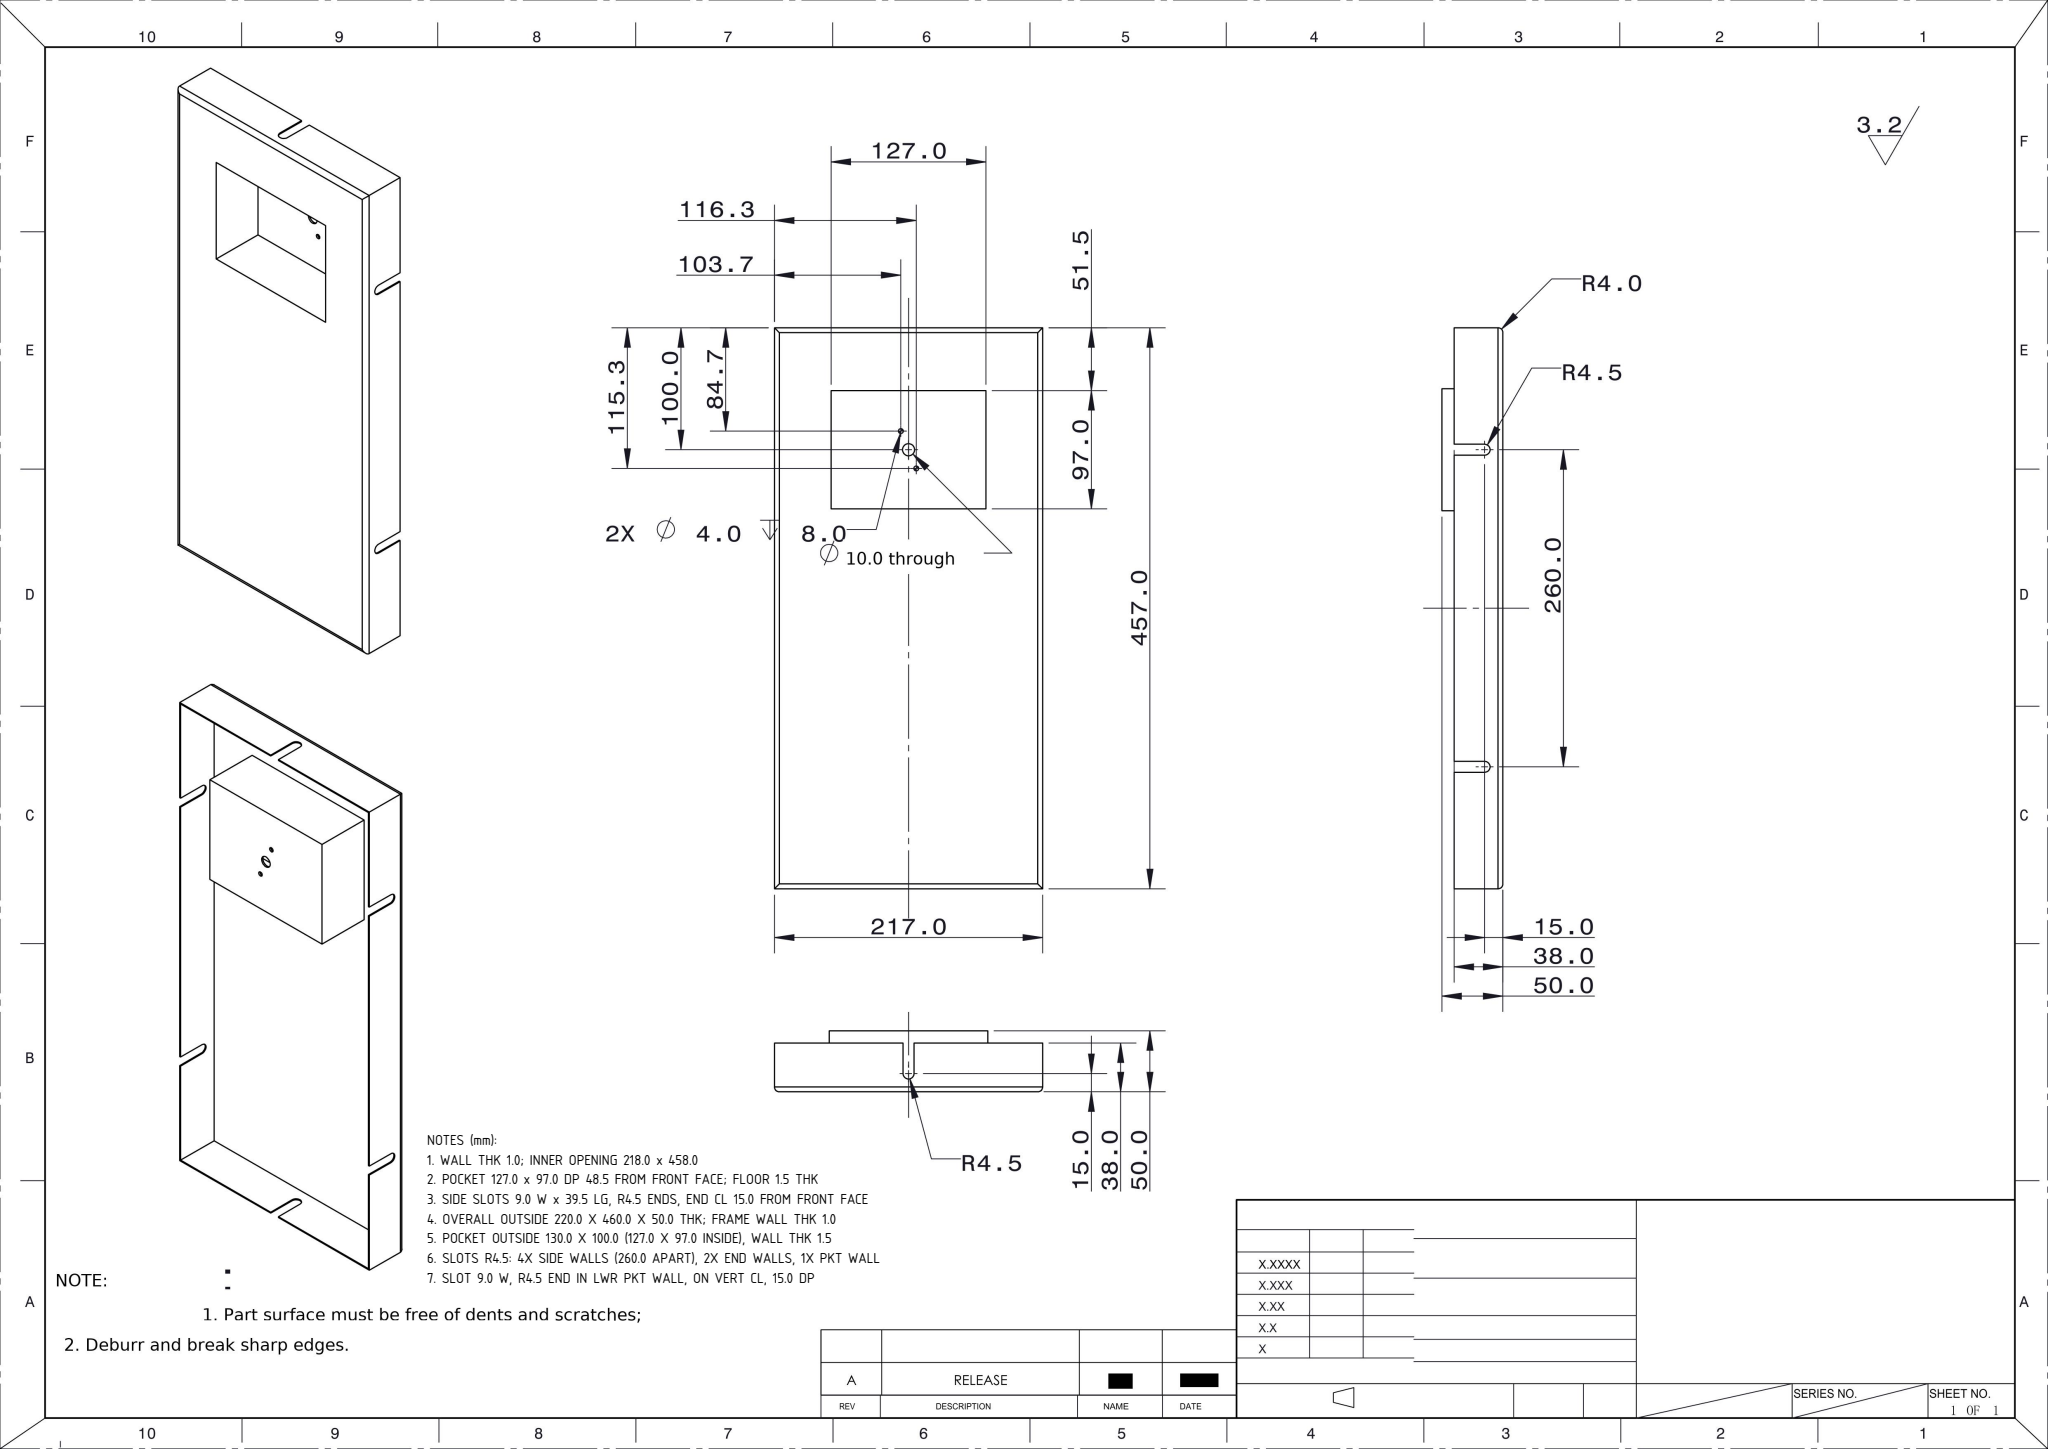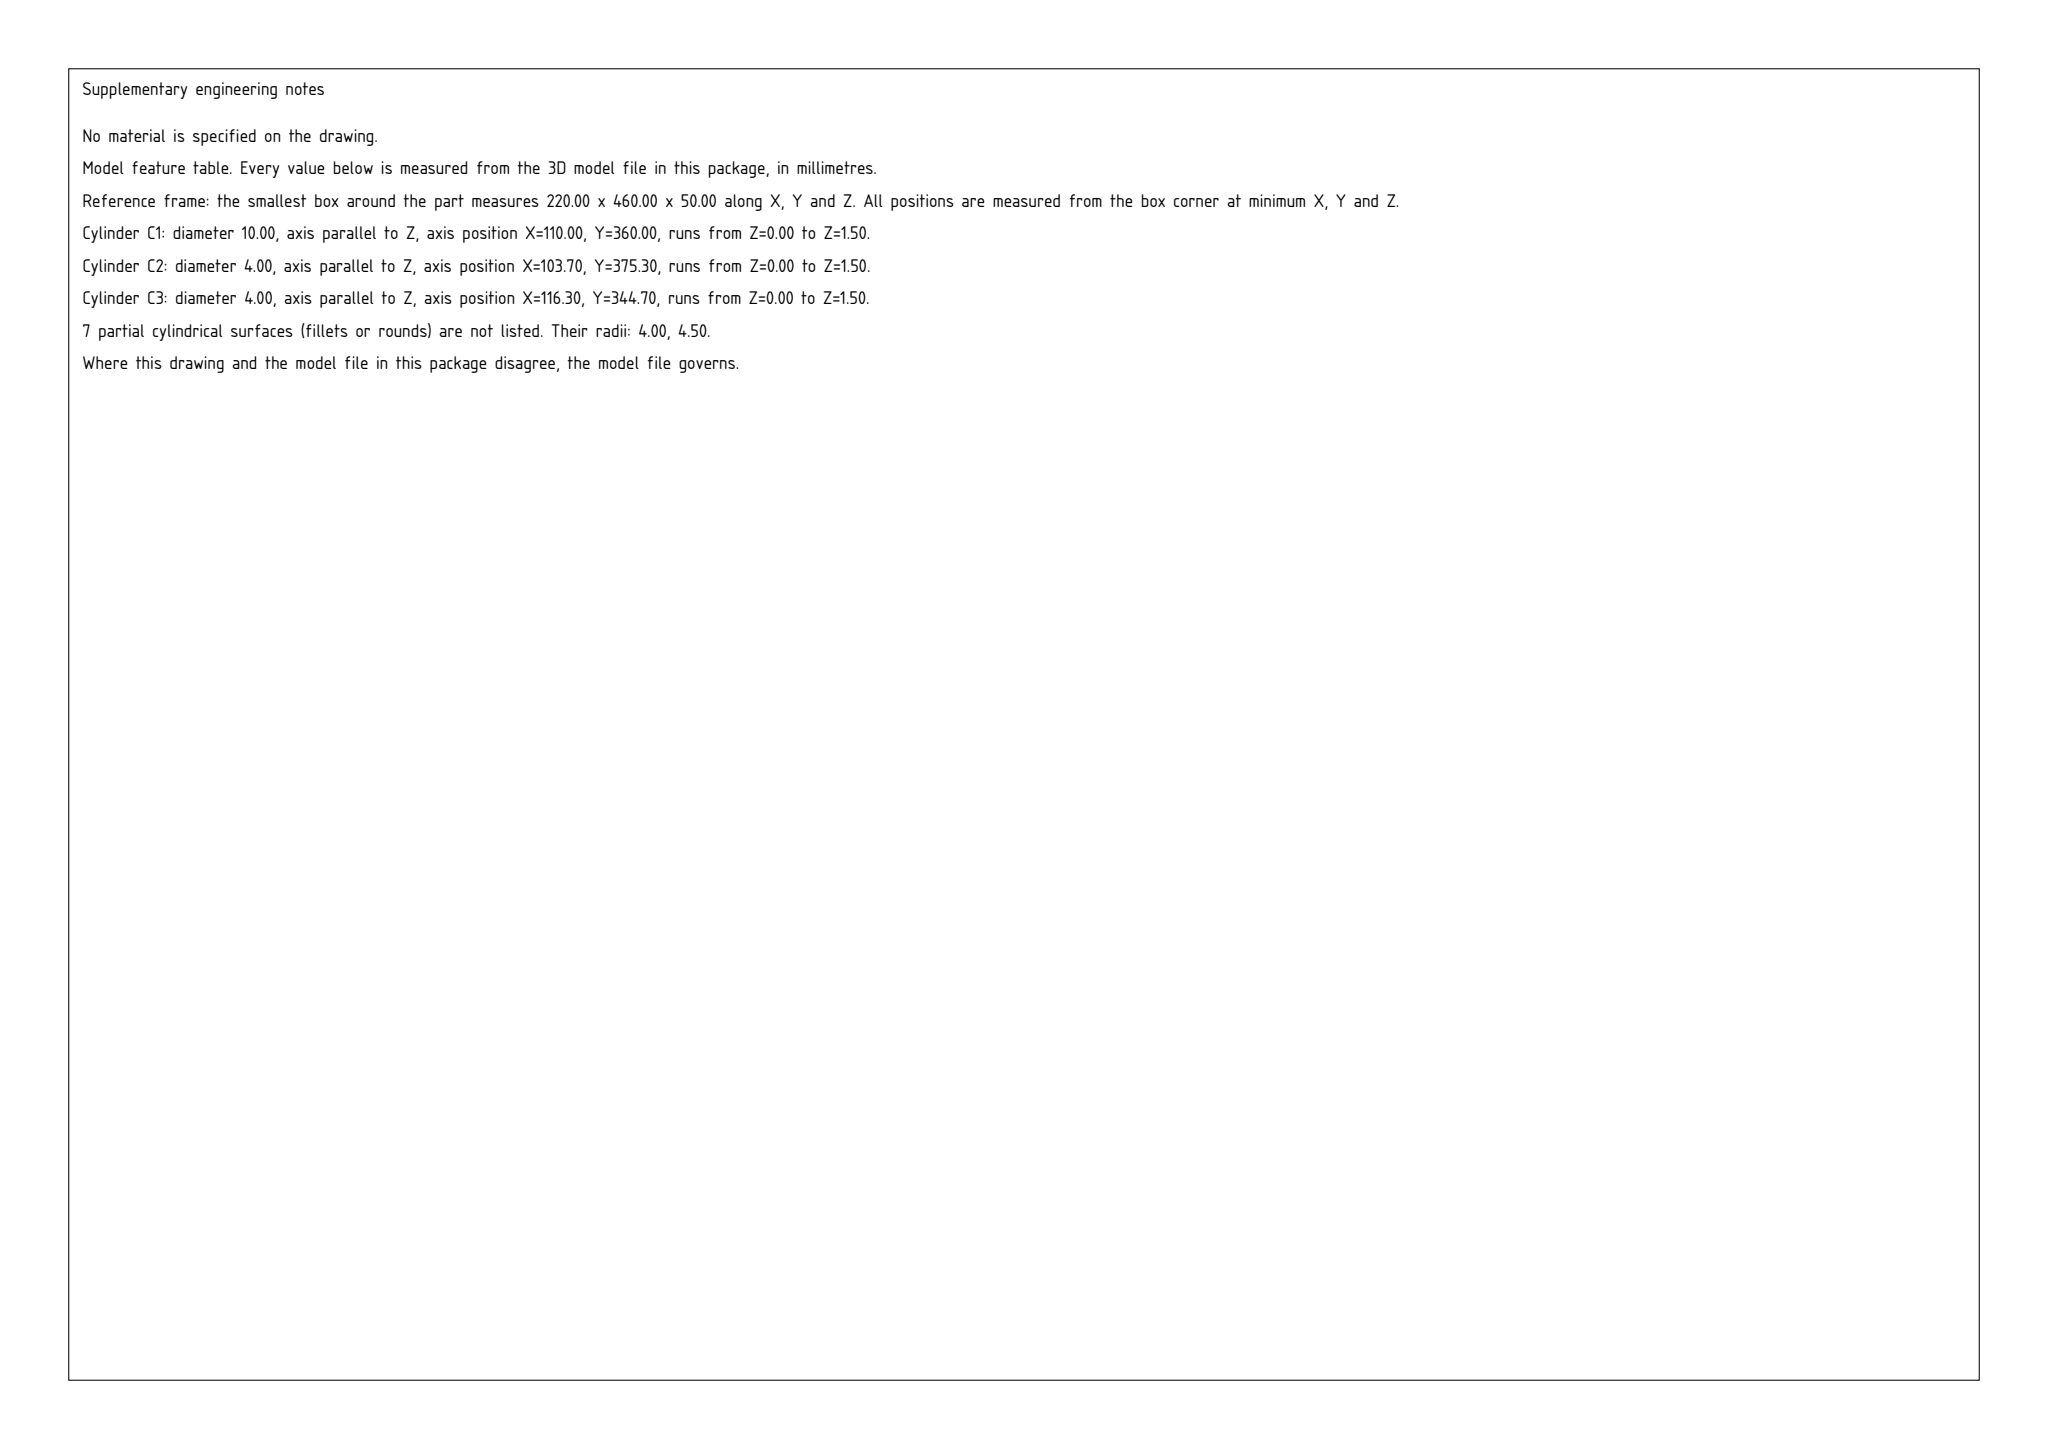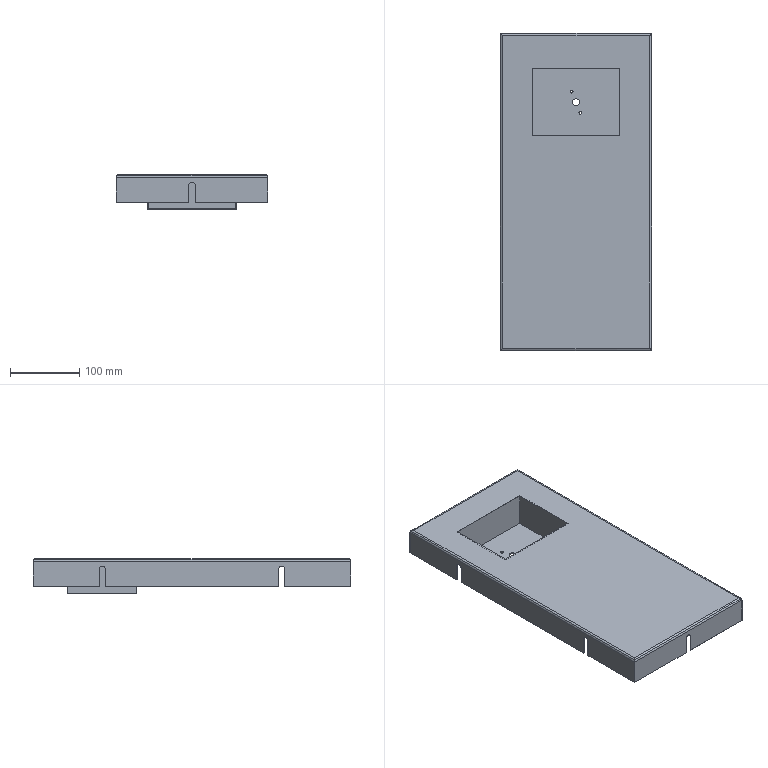Part | SolidWorks | mm | 1 solid | 55 faces | box 220 x 460 x 50 mm | volume 187271 mm3 | plane 38 | cylinder 17 | commonest cylinder face diameters 9 x7 4 x4 8 x4 10 x2
Drawing notes:
WALL THK 1.0; INNER OPENING 218.0 x 458.0 | from the solid: x-planes 0/1 & 219/220, y-planes 0/1 & 459/460 -> 1.0 wall, inner 218.0 x 458.0
POCKET 127.0 x 97.0 DP 48.5 FROM FRONT FACE; FLOOR 1.5 THK | from the solid: pocket inner x 46.5-173.5 (127.0), y 311.5-408.5 (97.0); floor z 0-1.5; front face z=50
SIDE SLOTS 9.0 W x 39.5 LG, R4.5 ENDS, END CL 15.0 FROM FRONT FACE | from the solid: O9 x-axis cyls at y=100 & y=360, z=35 thru 1.0 wall; y-planes 95.5/104.5; z 0-39.5; 50-35=15.0
OVERALL OUTSIDE 220.0 X 460.0 X 50.0 THK; FRAME WALL THK 1.0 | from the solid: bbox_xyz 220.0x460.0x50.0; x planes 0/1.0 & 219.0/220.0, y planes 0/1.0 & 459.0/460.0 give 1.0 wall
POCKET OUTSIDE 130.0 X 100.0 (127.0 X 97.0 INSIDE), WALL THK 1.5 | from the solid: x planes 45.0 & 175.0 (outside) vs 46.5 & 173.5 (inside); y planes 310.0 & 410.0 vs 311.5 & 408.5
SLOTS R4.5: 4X SIDE WALLS (260.0 APART), 2X END WALLS, 1X PKT WALL | from the solid: dia 9.0 cyl len 1.0: x-axis @ y=100 (x2) and y=360 (x2), z=35; y-axis @ x=110, z=35 (x3)
SLOT 9.0 W, R4.5 END IN LWR PKT WALL, ON VERT CL, 15.0 DP | from the solid: Cyl dia 9.0, axis y, at x=110.0 (bbox width 220 -> vert CL), z=35.0 (=15.0 from z=50 face), len 1.0; y-normal pocket wall planes y=310.0/311.5; slot flats y=95.5/104.5 & 355.5/364.5 confirm 9.0 wide slots with R4.5 ends
build123d program:
from build123d import *

# Parameters (mm, degrees)
SKETCH1_W                     = 220
SKETCH1_H                     = 460
BOSS_EXTRUDE1_DEPTH           = 40
SHELL1_T                      = -1
FILLET1_R                     = 4
SKETCH5_R                     = 10
SKETCH5_R_2                   = 2.5
CUT_EXTRUDE3_DEPTH            = 1106.462
SKETCH6_W                     = 130
SKETCH6_H                     = 100
BOSS_EXTRUDE2_DEPTH           = 50
SKETCH7_W                     = 127
SKETCH7_H                     = 97
CUT_EXTRUDE4_DEPTH            = 48.5
SKETCH8_R                     = 5
CUT_EXTRUDE5_DEPTH            = 1106.838
SIZE_MM_DOWEL_PIN_HOLE2_D     = 4
SIZE_MM_DOWEL_PIN_HOLE2_DEPTH = 8
SIZE_MM_DOWEL_PIN_HOLE2_TIP   = 1.202
CUT_EXTRUDE6_REACH            = 832.786
CUT_EXTRUDE7_REACH            = 893.807
CUT_EXTRUDE8_REACH            = 893.807
CUT_EXTRUDE9_REACH            = 832.786


with BuildPart() as part:
    # Sketch1 → Boss-Extrude1 (new body)
    with BuildSketch(Plane.XY):
        with Locations((580.004, 632.797)):
            Rectangle(SKETCH1_W, SKETCH1_H)
    extrude(amount=-BOSS_EXTRUDE1_DEPTH)

    # Shell1
    shell1_openings = [part.faces().sort_by_distance(p)[0] for p in [
        (580.004, 632.797, -40),
    ]]
    offset(amount=SHELL1_T, openings=shell1_openings, kind=Kind.INTERSECTION)

    # Fillet1
    fillet1_edges = [part.edges().sort_by_distance(p)[0] for p in [
        (580.004, 862.797, 0),
        (690.004, 632.797, 0),
        (580.004, 402.797, 0),
        (470.004, 632.797, 0),
    ]]
    fillet(fillet1_edges, radius=FILLET1_R)

    # Sketch5 → Cut-Extrude3 (cut, through all)
    with BuildSketch(Plane(origin=(0, 0, -1), x_dir=(-1, 0, 0), z_dir=(0, 0, -1))):
        with Locations((-580.004, 762.797)):
            Circle(SKETCH5_R)
        with Locations((-556.004, 786.797)):
            Circle(SKETCH5_R_2)
        with Locations((-604.004, 786.797)):
            Circle(SKETCH5_R_2)
        with Locations((-604.004, 738.797)):
            Circle(SKETCH5_R_2)
        with Locations((-556.004, 738.797)):
            Circle(SKETCH5_R_2)
    extrude(amount=-CUT_EXTRUDE3_DEPTH, mode=Mode.SUBTRACT)

    # Sketch6 → Boss-Extrude2 (add)
    with BuildSketch(Plane.XY):
        with Locations((580.004, 762.797)):
            Rectangle(SKETCH6_W, SKETCH6_H)
    extrude(amount=-BOSS_EXTRUDE2_DEPTH)

    # Sketch7 → Cut-Extrude4 (cut)
    with BuildSketch(Plane.XY):
        with Locations((580.004, 762.797)):
            Rectangle(SKETCH7_W, SKETCH7_H)
    extrude(amount=-CUT_EXTRUDE4_DEPTH, mode=Mode.SUBTRACT)

    # Sketch8 → Cut-Extrude5 (cut, through all)
    with BuildSketch(Plane.XY.offset(-48.5)):
        with Locations((580.004, 762.797)):
            Circle(SKETCH8_R)
    extrude(amount=-CUT_EXTRUDE5_DEPTH, mode=Mode.SUBTRACT)

    # Size mm Dowel Pin Hole2
    with Locations(Plane(origin=(0, 0, -50), x_dir=(-1, 0, 0), z_dir=(0, 0, -1))):
        with Locations((-573.704, 778.097), (-586.304, 747.497)):
            Hole(SIZE_MM_DOWEL_PIN_HOLE2_D / 2, depth=SIZE_MM_DOWEL_PIN_HOLE2_DEPTH)
            with Locations((0, 0, -(SIZE_MM_DOWEL_PIN_HOLE2_DEPTH + SIZE_MM_DOWEL_PIN_HOLE2_TIP / 2))):  # 118° drill point
                Cone(0, SIZE_MM_DOWEL_PIN_HOLE2_D / 2, SIZE_MM_DOWEL_PIN_HOLE2_TIP, mode=Mode.SUBTRACT)

    # Sketch13 → Cut-Extrude6 (cut, up to next)
    with BuildSketch(Plane.XZ.offset(-402.797), mode=Mode.PRIVATE) as cut_extrude6_sk1:
        with BuildLine():
            Line((584.504, -15), (584.504, -45))
            ThreePointArc((584.504, -45), (580.004, -49.5), (575.504, -45))
            Line((575.504, -45), (575.504, -15))
            ThreePointArc((575.504, -15), (580.004, -10.5), (584.504, -15))
        make_face()
    cut_extrude6_tool1 = extrude(cut_extrude6_sk1.sketch, amount=-CUT_EXTRUDE6_REACH, mode=Mode.PRIVATE) & part.part
    add(cut_extrude6_tool1.solids().sort_by_distance((580.004, 402.797, -30))[0], mode=Mode.SUBTRACT)

    # Sketch14 → Cut-Extrude7 (cut, up to next)
    with BuildSketch(Plane.ZY.offset(-470.004), mode=Mode.PRIVATE) as cut_extrude7_sk1:
        with BuildLine():
            Line((-45, 767.297), (-15, 767.297))
            ThreePointArc((-15, 767.297), (-10.5, 762.797), (-15, 758.297))
            Line((-15, 758.297), (-45, 758.297))
            ThreePointArc((-45, 758.297), (-49.5, 762.797), (-45, 767.297))
        make_face()
    cut_extrude7_tool1 = extrude(cut_extrude7_sk1.sketch, amount=-CUT_EXTRUDE7_REACH, mode=Mode.PRIVATE) & part.part
    # Sketch14 → Cut-Extrude7 (cut, up to next)
    with BuildSketch(Plane.ZY.offset(-470.004), mode=Mode.PRIVATE) as cut_extrude7_sk2:
        with BuildLine():
            Line((-45, 498.297), (-15, 498.297))
            ThreePointArc((-15, 498.297), (-10.5, 502.797), (-15, 507.297))
            Line((-15, 507.297), (-45, 507.297))
            ThreePointArc((-45, 507.297), (-49.5, 502.797), (-45, 498.297))
        make_face()
    cut_extrude7_tool2 = extrude(cut_extrude7_sk2.sketch, amount=-CUT_EXTRUDE7_REACH, mode=Mode.PRIVATE) & part.part
    add(cut_extrude7_tool1.solids().sort_by_distance((470.004, 762.797, -30))[0], mode=Mode.SUBTRACT)
    add(cut_extrude7_tool2.solids().sort_by_distance((470.004, 502.797, -30))[0], mode=Mode.SUBTRACT)

    # Sketch15 → Cut-Extrude8 (cut, up to next)
    with BuildSketch(Plane(origin=(690.004, 0, 0), x_dir=(0, 0, -1), z_dir=(1, 0, 0)), mode=Mode.PRIVATE) as cut_extrude8_sk1:
        with BuildLine():
            Line((15, 767.297), (45, 767.297))
            ThreePointArc((45, 767.297), (49.5, 762.797), (45, 758.297))
            Line((45, 758.297), (15, 758.297))
            ThreePointArc((15, 758.297), (10.5, 762.797), (15, 767.297))
        make_face()
    cut_extrude8_tool1 = extrude(cut_extrude8_sk1.sketch, amount=-CUT_EXTRUDE8_REACH, mode=Mode.PRIVATE) & part.part
    # Sketch15 → Cut-Extrude8 (cut, up to next)
    with BuildSketch(Plane(origin=(690.004, 0, 0), x_dir=(0, 0, -1), z_dir=(1, 0, 0)), mode=Mode.PRIVATE) as cut_extrude8_sk2:
        with BuildLine():
            Line((15, 498.297), (45, 498.297))
            ThreePointArc((45, 498.297), (49.5, 502.797), (45, 507.297))
            Line((45, 507.297), (15, 507.297))
            ThreePointArc((15, 507.297), (10.5, 502.797), (15, 498.297))
        make_face()
    cut_extrude8_tool2 = extrude(cut_extrude8_sk2.sketch, amount=-CUT_EXTRUDE8_REACH, mode=Mode.PRIVATE) & part.part
    add(cut_extrude8_tool1.solids().sort_by_distance((690.004, 762.797, -30))[0], mode=Mode.SUBTRACT)
    add(cut_extrude8_tool2.solids().sort_by_distance((690.004, 502.797, -30))[0], mode=Mode.SUBTRACT)

    # Sketch16 → Cut-Extrude9 (cut, up to next)
    with BuildSketch(Plane(origin=(0, 862.797, 0), x_dir=(1, 0, 0), z_dir=(0, 1, 0)), mode=Mode.PRIVATE) as cut_extrude9_sk1:
        with BuildLine():
            Line((584.504, 45), (584.504, 15))
            ThreePointArc((584.504, 15), (580.004, 10.5), (575.504, 15))
            Line((575.504, 15), (575.504, 45))
            ThreePointArc((575.504, 45), (580.004, 49.5), (584.504, 45))
        make_face()
    cut_extrude9_tool1 = extrude(cut_extrude9_sk1.sketch, amount=-CUT_EXTRUDE9_REACH, mode=Mode.PRIVATE) & part.part
    add(cut_extrude9_tool1.solids().sort_by_distance((580.004, 862.797, -30))[0], mode=Mode.SUBTRACT)


solid = part.part